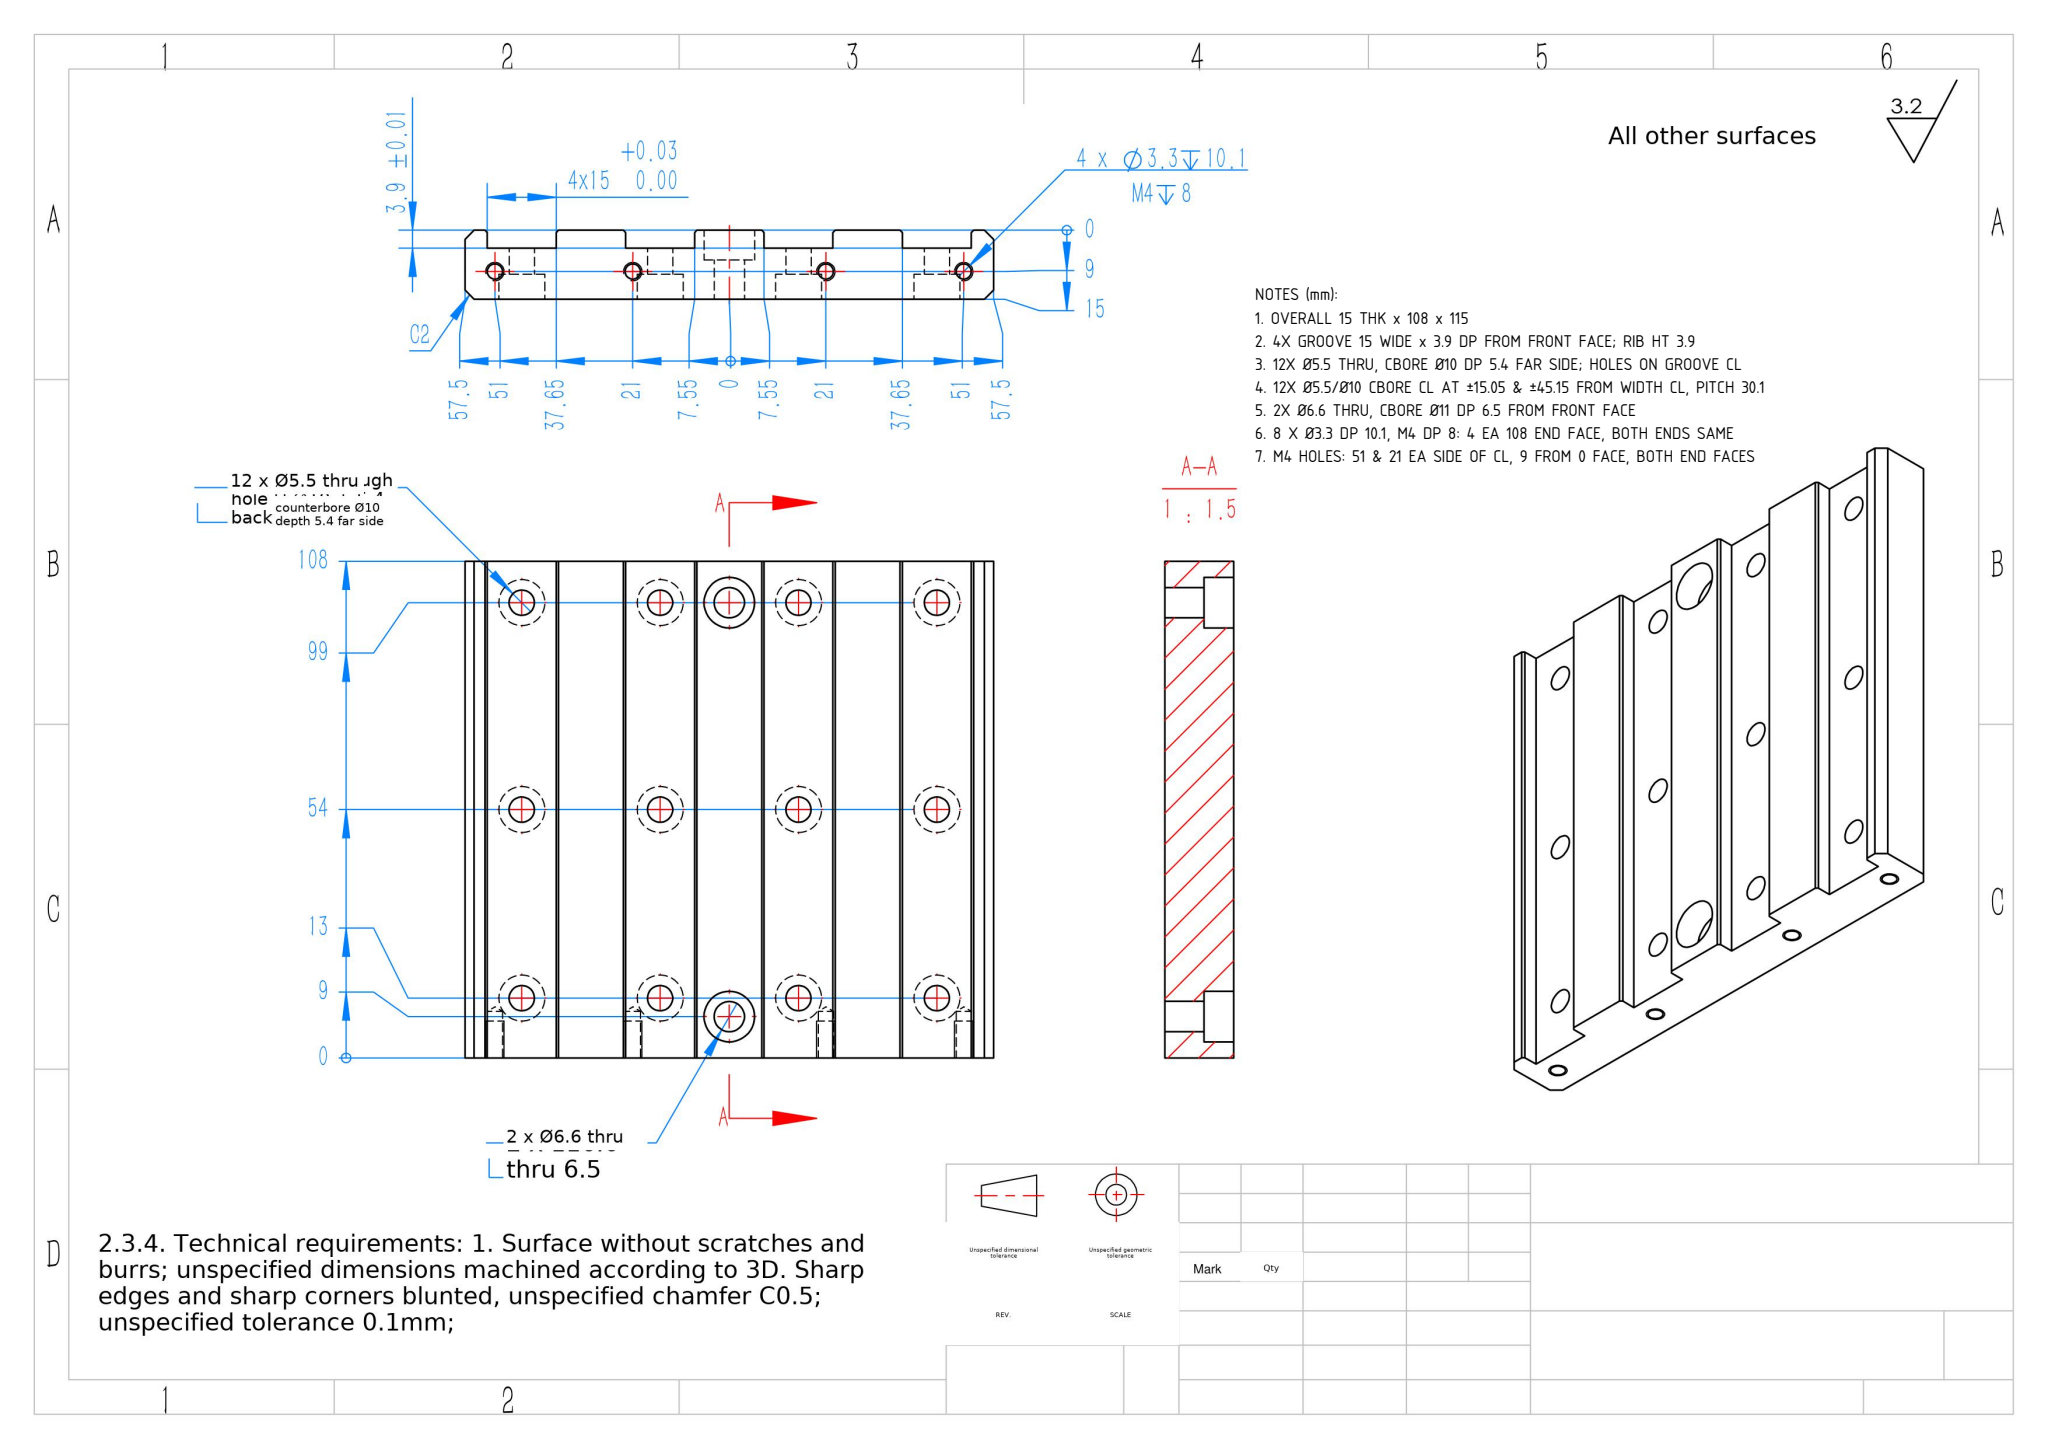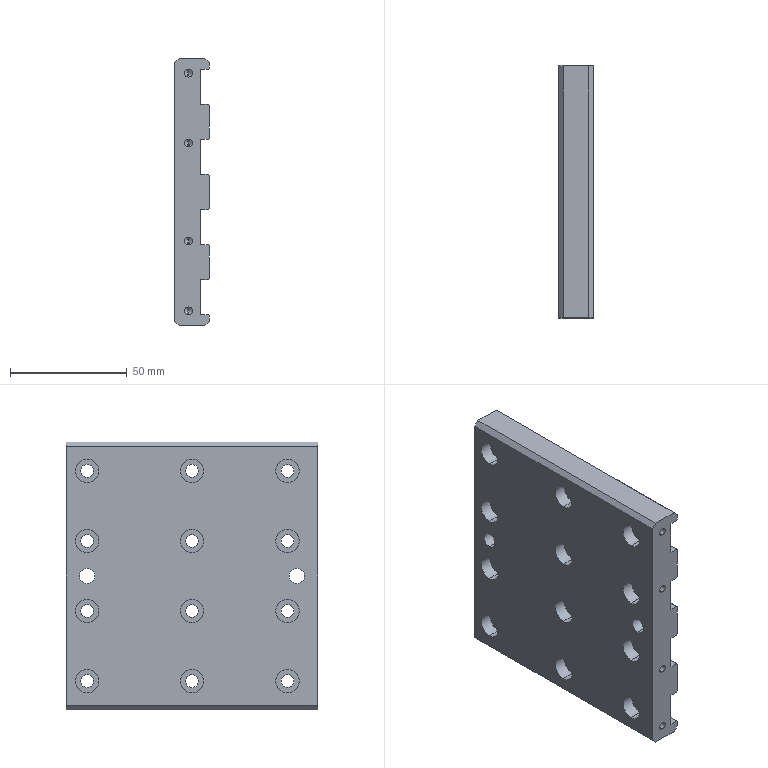Part | SolidWorks | mm | 1 solid | 120 faces | box 15 x 108 x 115 mm | volume 151168 mm3 | cylinder 64 | plane 48 | cone 8 | commonest cylinder face diameters 10 x24 5.5 x24 3.3 x8 11 x4 6.6 x4
Drawing notes:
OVERALL 15 THK x 108 x 115 | from the solid: bbox_xyz 15.0 x 108.0 x 115.0
4X GROOVE 15 WIDE x 3.9 DP FROM FRONT FACE; RIB HT 3.9 | from the solid: x-planes: front face 15.0, groove floors x=11.1 (qty 4); 15-11.1=3.9
12X Ø5.5 THRU, CBORE Ø10 DP 5.4 FAR SIDE; HOLES ON GROOVE CL | from the solid: Ø5.5 x-axis len 5.7 and Ø10 len 5.4 at same z; groove edges 7.55/37.65 from CL give groove CL = hole CL
12X Ø5.5/Ø10 CBORE CL AT ±15.05 & ±45.15 FROM WIDTH CL, PITCH 30.1 | from the solid: holes at z=12.35, 42.45, 72.55, 102.65; bbox z=115 so CL=57.5; spacing 42.45-12.35=30.1
2X Ø6.6 THRU, CBORE Ø11 DP 6.5 FROM FRONT FACE | from the solid: Ø6.6 x-axis len 8.5 at y=9 & y=99, z=57.5; Ø11 len 6.5 -> bore floor x=8.5, front face x=15
8 X Ø3.3 DP 10.1, M4 DP 8: 4 EA 108 END FACE, BOTH ENDS SAME | from the solid: cylinders Ø3.3 axis Y, L=10.1, at z=6.5/36.5/78.5/108.5, count 2 each (y=0 and y=108 faces) = 8 holes; cones 118° ref dia 3.3 count 8
M4 HOLES: 51 & 21 EA SIDE OF CL, 9 FROM 0 FACE, BOTH END FACES | from the solid: z=6.5/36.5/78.5/108.5 vs part z 0-115 (CL 57.5) gives ±51 & ±21; x=6.0 of 15 thk = 9 from x=15 (0 datum) face
build123d program:
from build123d import *

# Parameters (mm, degrees)
SKETCH1_W                                       = 115
SKETCH1_H                                       = 108
BOSS_EXTRUDE1_DEPTH                             = 7.5
SKETCH2_W                                       = 15
SKETCH2_H                                       = 108
CUT_EXTRUDE1_DEPTH                              = 3.9
M5_HEX_SOCKET_HEAD_CAP_SCREW_CBORE2_D           = 5.5
M5_HEX_SOCKET_HEAD_CAP_SCREW_CBORE2_CBORE_D     = 10
M5_HEX_SOCKET_HEAD_CAP_SCREW_CBORE2_CBORE_DEPTH = 5.4
M6_HEX_SOCKET_HEAD_CAP_SCREW_CBORE1_D           = 6.6
M6_HEX_SOCKET_HEAD_CAP_SCREW_CBORE1_CBORE_D     = 11
M6_HEX_SOCKET_HEAD_CAP_SCREW_CBORE1_CBORE_DEPTH = 6.5
M4_TAPPED_HOLE1_D                               = 3.3
M4_TAPPED_HOLE1_DEPTH                           = 10.1
M4_TAPPED_HOLE1_TIP                             = 0.9914
CHAMFER1_SIZE                                   = 0.5
CHAMFER2_SIZE                                   = 2
CHAMFER3_SIZE                                   = 2


with BuildPart() as part:
    # Sketch1 → Boss-Extrude1 (new, symmetric)
    with BuildSketch(Plane(origin=(0, 0, 0), x_dir=(0, 0, -1), z_dir=(1, 0, 0))):
        Rectangle(SKETCH1_W, SKETCH1_H)
    extrude(amount=BOSS_EXTRUDE1_DEPTH, both=True)

    # Sketch2 → Cut-Extrude1 (cut)
    with BuildSketch(Plane(origin=(7.5, 0, 0), x_dir=(0, 0, -1), z_dir=(1, 0, 0))):
        with Locations((15.05, 0)):
            Rectangle(SKETCH2_W, SKETCH2_H)
        with Locations((-15.05, 0)):
            Rectangle(SKETCH2_W, SKETCH2_H)
        with Locations((45.15, 0)):
            Rectangle(SKETCH2_W, SKETCH2_H)
        with Locations((-45.15, 0)):
            Rectangle(SKETCH2_W, SKETCH2_H)
    extrude(amount=-CUT_EXTRUDE1_DEPTH, mode=Mode.SUBTRACT)

    # M5 Hex Socket Head Cap Screw CBORE2 (through all)
    with Locations(Plane.ZY.offset(7.5)):
        with Locations((-45.15, 45), (-45.15, 0), (-45.15, -41), (-15.05, 45), (-15.05, 0), (-15.05, -41), (15.05, -41), (15.05, 0), (15.05, 45), (45.15, 45), (45.15, 0), (45.15, -41)):
            CounterBoreHole(M5_HEX_SOCKET_HEAD_CAP_SCREW_CBORE2_D / 2, M5_HEX_SOCKET_HEAD_CAP_SCREW_CBORE2_CBORE_D / 2, M5_HEX_SOCKET_HEAD_CAP_SCREW_CBORE2_CBORE_DEPTH)

    # M6 Hex Socket Head Cap Screw CBORE1 (through all)
    with Locations(Plane(origin=(7.5, 0, 0), x_dir=(0, 0, -1), z_dir=(1, 0, 0))):
        with Locations((0, 45), (0, -45)):
            CounterBoreHole(M6_HEX_SOCKET_HEAD_CAP_SCREW_CBORE1_D / 2, M6_HEX_SOCKET_HEAD_CAP_SCREW_CBORE1_CBORE_D / 2, M6_HEX_SOCKET_HEAD_CAP_SCREW_CBORE1_CBORE_DEPTH)

    # M4 Tapped Hole1
    with Locations(Plane(origin=(0, -54, 0), x_dir=(-1, 0, 0), z_dir=(0, -1, 0))):
        with Locations((1.5, -21), (1.5, 21), (1.5, -51), (1.5, 51)):
            Hole(M4_TAPPED_HOLE1_D / 2, depth=M4_TAPPED_HOLE1_DEPTH)
            with Locations((0, 0, -(M4_TAPPED_HOLE1_DEPTH + M4_TAPPED_HOLE1_TIP / 2))):  # 118° drill point
                Cone(0, M4_TAPPED_HOLE1_D / 2, M4_TAPPED_HOLE1_TIP, mode=Mode.SUBTRACT)

    # Chamfer1
    chamfer1_edges = [part.edges().sort_by_distance(p)[0] for p in [
        (7.5, 0, 52.65),
        (7.5, 0, 37.65),
        (7.5, 0, -52.65),
        (7.5, 0, -37.65),
        (7.5, 0, 7.55),
        (7.5, 0, 22.55),
        (7.5, 0, -22.55),
        (7.5, 0, -7.55),
    ]]
    chamfer(chamfer1_edges, length=CHAMFER1_SIZE)

    # Chamfer2
    chamfer2_edges = [part.edges().sort_by_distance(p)[0] for p in [
        (-7.5, 0, 57.5),
        (-7.5, 0, -57.5),
    ]]
    chamfer(chamfer2_edges, length=CHAMFER2_SIZE)

    # Chamfer3
    chamfer3_edges = [part.edges().sort_by_distance(p)[0] for p in [
        (7.5, 0, 57.5),
        (7.5, 0, -57.5),
    ]]
    chamfer(chamfer3_edges, length=CHAMFER3_SIZE)


solid = part.part